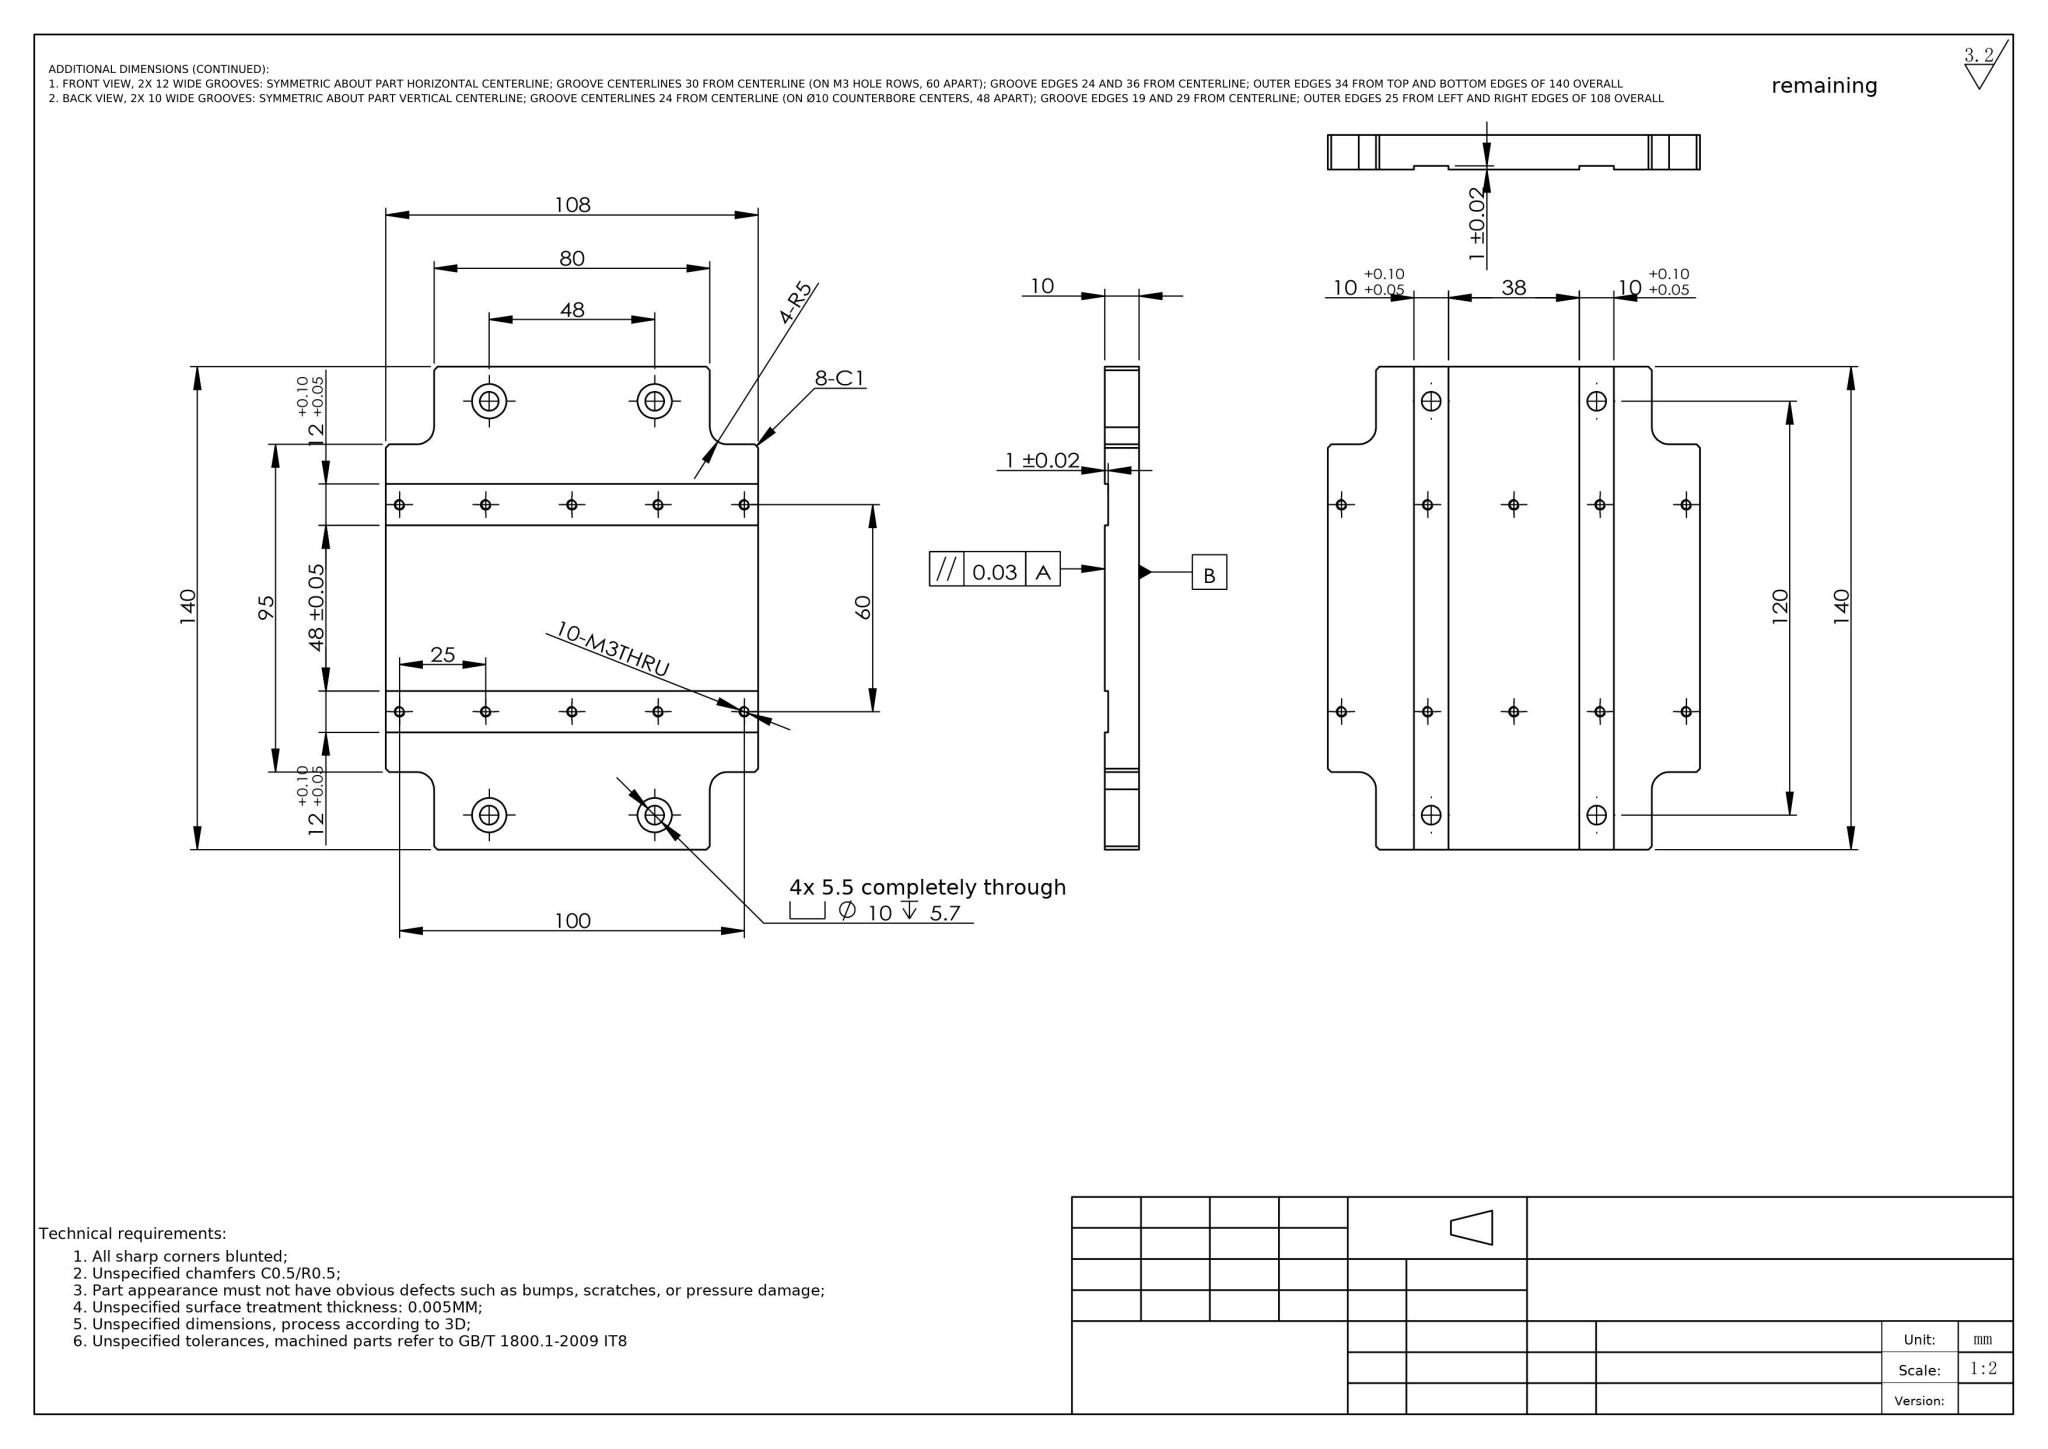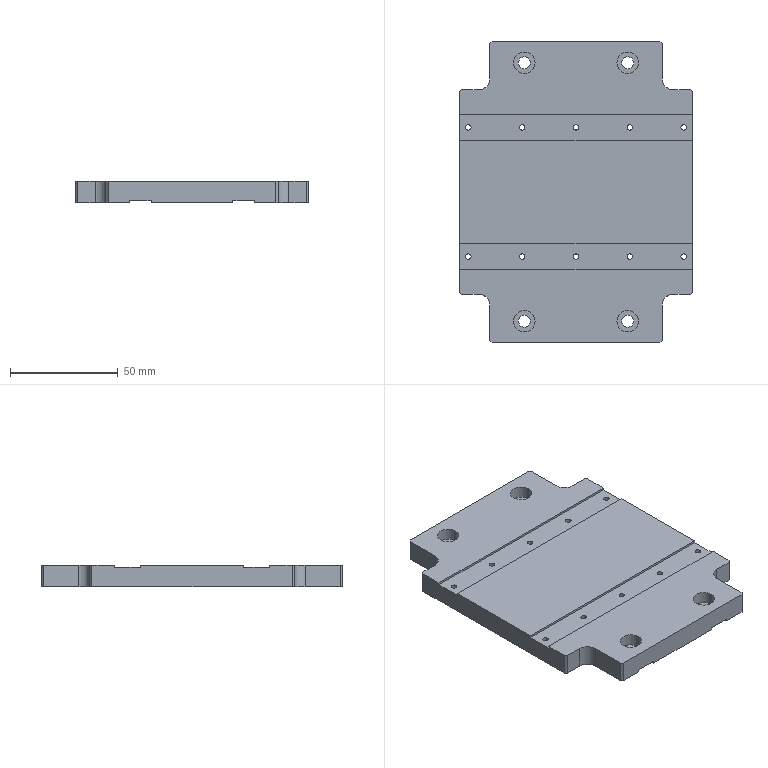Part | NX | mm | 1 solid | 82 faces | box 108 x 140 x 10 mm | volume 130856 mm3 | plane 42 | cylinder 40 | commonest cylinder face diameters 2.5 x20 10 x12 5.5 x8